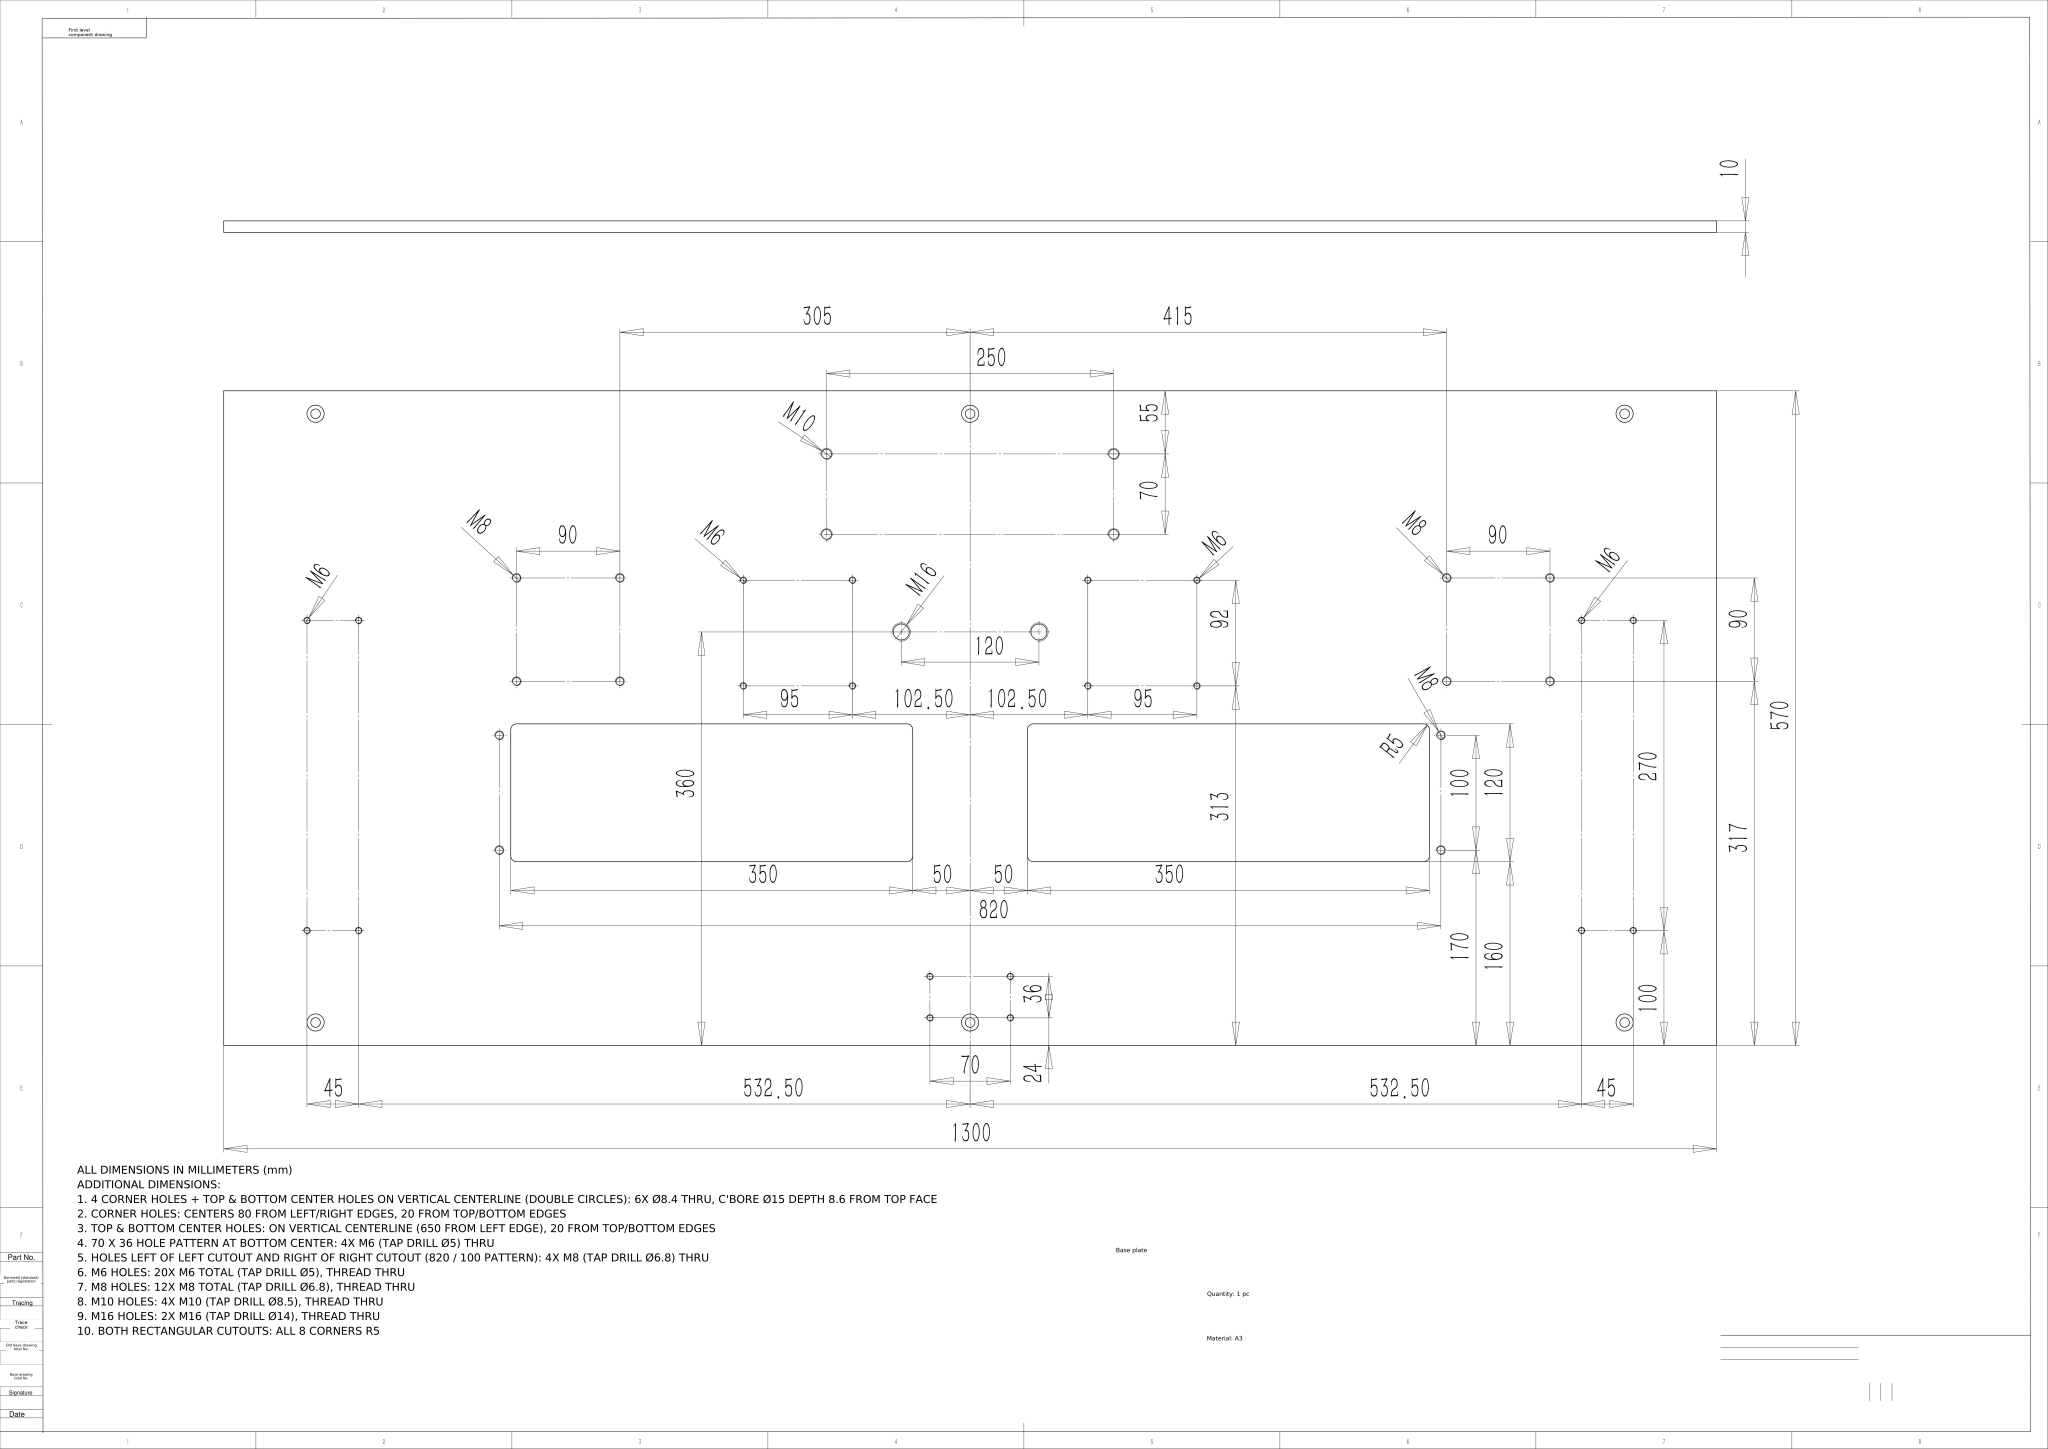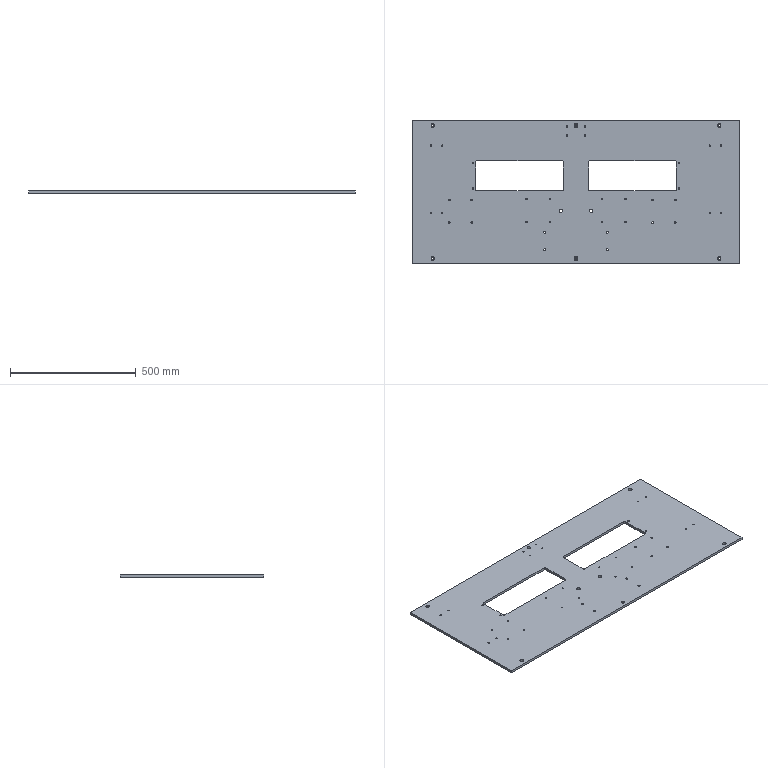Part | NX | mm | 1 solid | 128 faces | box 1300 x 570 x 10 mm | volume 6547212 mm3 | cylinder 108 | plane 20 | commonest cylinder face diameters 5 x40 6.8 x24 15 x12 8.4 x12 8.5 x8 10 x8 14 x4